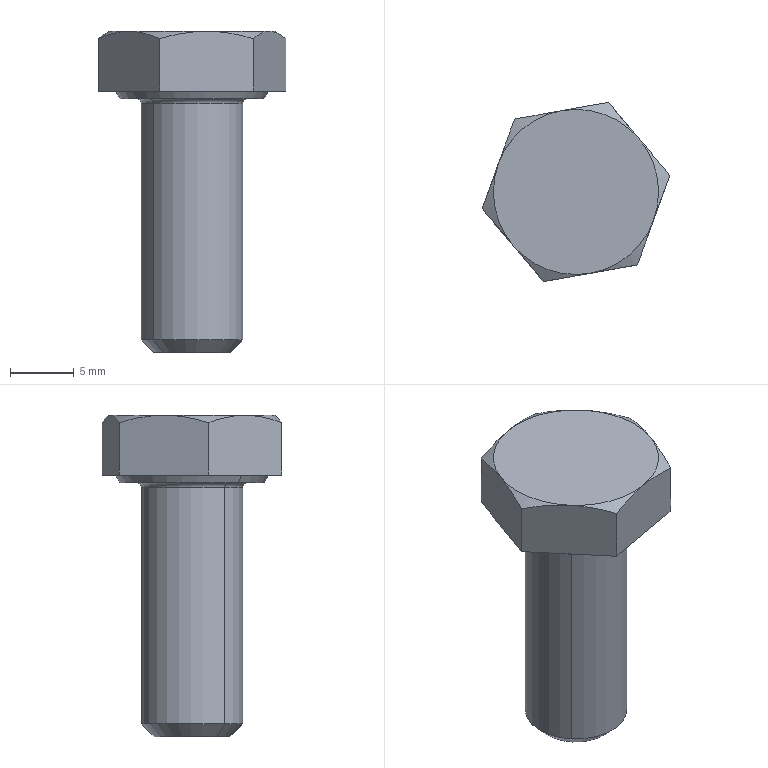Component | SolidWorks | GB_T5781-2000[HexHeadBoltFullThreadGradeCM8_20]-2 | 1 solid | 24 faces | box 14.78 x 14.12 x 25.3 mm | volume 1745 mm3 | cone 10 | plane 10 | cylinder 2 | torus 2 | commonest cylinder face diameters 8 x2
STEP:
#1=COLOUR_RGB('',0.7922,0.8196,0.9333);
#2=FILL_AREA_STYLE_COLOUR('',#1);
#3=FILL_AREA_STYLE('',(#2));
#4=SURFACE_STYLE_FILL_AREA(#3);
#5=SURFACE_SIDE_STYLE('',(#4));
#6=SURFACE_STYLE_USAGE(.BOTH.,#5);
#7=PRESENTATION_STYLE_ASSIGNMENT((#6));
#8=CARTESIAN_POINT('',(19.172,-21.185,97.148));
#9=VERTEX_POINT('',#8);
#10=CARTESIAN_POINT('',(18.931,-21.388,97.148));
#11=VERTEX_POINT('',#10);
#12=CARTESIAN_POINT('',(19.052,-21.287,97.148));
#13=DIRECTION('',(-0.,-0.,1.));
#14=DIRECTION('',(0.7644,0.6448,0.));
#15=AXIS2_PLACEMENT_3D('',#12,#13,#14);
#16=CIRCLE('',#15,0.1575);
#17=EDGE_CURVE('',#9,#11,#16,.T.);
#18=ORIENTED_EDGE('',*,*,#17,.F.);
#19=CARTESIAN_POINT('',(19.172,-21.185,96.416));
#20=VERTEX_POINT('',#19);
#21=CARTESIAN_POINT('',(19.172,-21.185,97.373));
#22=DIRECTION('',(0.,0.,-1.));
#23=VECTOR('',#22,39.37);
#24=LINE('',#21,#23);
#25=EDGE_CURVE('',#9,#20,#24,.T.);
#26=ORIENTED_EDGE('',*,*,#25,.T.);
#27=CARTESIAN_POINT('',(18.931,-21.388,96.416));
#28=VERTEX_POINT('',#27);
#29=CARTESIAN_POINT('',(19.052,-21.287,96.416));
#30=DIRECTION('',(-0.,-0.,1.));
#31=DIRECTION('',(-0.7644,-0.6448,-0.));
#32=AXIS2_PLACEMENT_3D('',#29,#30,#31);
#33=CIRCLE('',#32,0.1575);
#34=EDGE_CURVE('',#20,#28,#33,.T.);
#35=ORIENTED_EDGE('',*,*,#34,.T.);
#36=CARTESIAN_POINT('',(18.931,-21.388,97.373));
#37=DIRECTION('',(0.,0.,-1.));
#38=VECTOR('',#37,39.37);
#39=LINE('',#36,#38);
#40=EDGE_CURVE('',#11,#28,#39,.T.);
#41=ORIENTED_EDGE('',*,*,#40,.F.);
#42=EDGE_LOOP('',(#18,#26,#35,#41));
#43=FACE_OUTER_BOUND('',#42,.T.);
#44=CARTESIAN_POINT('',(19.052,-21.287,97.373));
#45=DIRECTION('',(0.,0.,-1.));
#46=DIRECTION('',(-0.7644,-0.6448,-0.));
#47=AXIS2_PLACEMENT_3D('',#44,#45,#46);
#48=CYLINDRICAL_SURFACE('',#47,0.1575);
#49=ADVANCED_FACE('',(#43),#48,.T.);
#50=CARTESIAN_POINT('',(18.962,-21.363,96.377));
#51=VERTEX_POINT('',#50);
#52=CARTESIAN_POINT('',(19.142,-21.21,96.377));
#53=VERTEX_POINT('',#52);
#54=CARTESIAN_POINT('',(19.052,-21.287,96.377));
#55=DIRECTION('',(0.,0.,-1.));
#56=DIRECTION('',(-0.7644,-0.6448,-0.));
#57=AXIS2_PLACEMENT_3D('',#54,#55,#56);
#58=CIRCLE('',#57,0.1181);
#59=EDGE_CURVE('',#51,#53,#58,.T.);
#60=ORIENTED_EDGE('',*,*,#59,.F.);
#61=CARTESIAN_POINT('',(18.962,-21.363,96.377));
#62=DIRECTION('',(-0.5405,-0.4559,0.7071));
#63=VECTOR('',#62,39.37);
#64=LINE('',#61,#63);
#65=EDGE_CURVE('',#51,#28,#64,.T.);
#66=ORIENTED_EDGE('',*,*,#65,.T.);
#67=ORIENTED_EDGE('',*,*,#34,.F.);
#68=CARTESIAN_POINT('',(19.142,-21.21,96.377));
#69=DIRECTION('',(0.5405,0.4559,0.7071));
#70=VECTOR('',#69,39.37);
#71=LINE('',#68,#70);
#72=EDGE_CURVE('',#53,#20,#71,.T.);
#73=ORIENTED_EDGE('',*,*,#72,.F.);
#74=EDGE_LOOP('',(#60,#66,#67,#73));
#75=FACE_OUTER_BOUND('',#74,.T.);
#76=CARTESIAN_POINT('',(19.052,-21.287,96.377));
#77=DIRECTION('',(-0.,-0.,1.));
#78=DIRECTION('',(0.7644,0.6448,0.));
#79=AXIS2_PLACEMENT_3D('',#76,#77,#78);
#80=CONICAL_SURFACE('',#79,0.1181,0.7854);
#81=ADVANCED_FACE('',(#75),#80,.T.);
#82=CARTESIAN_POINT('',(18.919,-21.398,97.164));
#83=VERTEX_POINT('',#82);
#84=CARTESIAN_POINT('',(19.184,-21.175,97.164));
#85=VERTEX_POINT('',#84);
#86=CARTESIAN_POINT('',(19.052,-21.287,97.164));
#87=DIRECTION('',(-0.,-0.,1.));
#88=DIRECTION('',(0.7644,0.6448,0.));
#89=AXIS2_PLACEMENT_3D('',#86,#87,#88);
#90=CIRCLE('',#89,0.1732);
#91=EDGE_CURVE('',#83,#85,#90,.T.);
#92=ORIENTED_EDGE('',*,*,#91,.F.);
#93=CARTESIAN_POINT('',(18.919,-21.398,97.148));
#94=DIRECTION('',(-0.6448,0.7644,0.));
#95=DIRECTION('',(-0.7644,-0.6448,0.));
#96=AXIS2_PLACEMENT_3D('',#93,#94,#95);
#97=CIRCLE('',#96,0.01575);
#98=EDGE_CURVE('',#83,#11,#97,.T.);
#99=ORIENTED_EDGE('',*,*,#98,.T.);
#100=CARTESIAN_POINT('',(19.052,-21.287,97.148));
#101=DIRECTION('',(-0.,-0.,1.));
#102=DIRECTION('',(0.7644,0.6448,0.));
#103=AXIS2_PLACEMENT_3D('',#100,#101,#102);
#104=CIRCLE('',#103,0.1575);
#105=EDGE_CURVE('',#11,#9,#104,.T.);
#106=ORIENTED_EDGE('',*,*,#105,.T.);
#107=CARTESIAN_POINT('',(19.184,-21.175,97.148));
#108=DIRECTION('',(0.6448,-0.7644,-0.));
#109=DIRECTION('',(0.7644,0.6448,0.));
#110=AXIS2_PLACEMENT_3D('',#107,#108,#109);
#111=CIRCLE('',#110,0.01575);
#112=EDGE_CURVE('',#85,#9,#111,.T.);
#113=ORIENTED_EDGE('',*,*,#112,.F.);
#114=EDGE_LOOP('',(#92,#99,#106,#113));
#115=FACE_OUTER_BOUND('',#114,.T.);
#116=CARTESIAN_POINT('',(19.052,-21.287,97.148));
#117=DIRECTION('',(-0.,-0.,1.));
#118=DIRECTION('',(0.7644,0.6448,0.));
#119=AXIS2_PLACEMENT_3D('',#116,#117,#118);
#120=TOROIDAL_SURFACE('',#119,0.1732,0.01575);
#121=ADVANCED_FACE('',(#115),#120,.F.);
#122=CARTESIAN_POINT('',(19.223,-21.143,97.164));
#123=VERTEX_POINT('',#122);
#124=CARTESIAN_POINT('',(18.881,-21.431,97.164));
#125=VERTEX_POINT('',#124);
#126=CARTESIAN_POINT('',(19.052,-21.287,97.164));
#127=DIRECTION('',(-0.,-0.,1.));
#128=DIRECTION('',(0.7644,0.6448,0.));
#129=AXIS2_PLACEMENT_3D('',#126,#127,#128);
#130=CIRCLE('',#129,0.2235);
#131=EDGE_CURVE('',#123,#125,#130,.T.);
#132=ORIENTED_EDGE('',*,*,#131,.T.);
#133=CARTESIAN_POINT('',(18.871,-21.44,97.188));
#134=VERTEX_POINT('',#133);
#135=CARTESIAN_POINT('',(18.871,-21.44,97.188));
#136=DIRECTION('',(-0.3822,-0.3224,0.866));
#137=VECTOR('',#136,39.37);
#138=LINE('',#135,#137);
#139=EDGE_CURVE('',#125,#134,#138,.T.);
#140=ORIENTED_EDGE('',*,*,#139,.T.);
#141=CARTESIAN_POINT('',(19.233,-21.134,97.188));
#142=VERTEX_POINT('',#141);
#143=CARTESIAN_POINT('',(19.052,-21.287,97.188));
#144=DIRECTION('',(-0.,-0.,1.));
#145=DIRECTION('',(0.7644,0.6448,0.));
#146=AXIS2_PLACEMENT_3D('',#143,#144,#145);
#147=CIRCLE('',#146,0.2372);
#148=EDGE_CURVE('',#142,#134,#147,.T.);
#149=ORIENTED_EDGE('',*,*,#148,.F.);
#150=CARTESIAN_POINT('',(19.233,-21.134,97.188));
#151=DIRECTION('',(0.3822,0.3224,0.866));
#152=VECTOR('',#151,39.37);
#153=LINE('',#150,#152);
#154=EDGE_CURVE('',#123,#142,#153,.T.);
#155=ORIENTED_EDGE('',*,*,#154,.F.);
#156=EDGE_LOOP('',(#132,#140,#149,#155));
#157=FACE_OUTER_BOUND('',#156,.T.);
#158=CARTESIAN_POINT('',(19.052,-21.287,97.188));
#159=DIRECTION('',(-0.,-0.,1.));
#160=DIRECTION('',(0.7644,0.6448,0.));
#161=AXIS2_PLACEMENT_3D('',#158,#159,#160);
#162=CONICAL_SURFACE('',#161,0.2372,0.5236);
#163=ADVANCED_FACE('',(#157),#162,.T.);
#164=ORIENTED_EDGE('',*,*,#131,.F.);
#165=CARTESIAN_POINT('',(19.052,-21.287,97.164));
#166=DIRECTION('',(-0.,-0.,1.));
#167=DIRECTION('',(0.7644,0.6448,0.));
#168=AXIS2_PLACEMENT_3D('',#165,#166,#167);
#169=CIRCLE('',#168,0.2235);
#170=EDGE_CURVE('',#125,#123,#169,.T.);
#171=ORIENTED_EDGE('',*,*,#170,.F.);
#172=EDGE_LOOP('',(#164,#171));
#173=FACE_OUTER_BOUND('',#172,.T.);
#174=CARTESIAN_POINT('',(19.052,-21.287,97.164));
#175=DIRECTION('',(-0.,-0.,1.));
#176=DIRECTION('',(0.7644,0.6448,0.));
#177=AXIS2_PLACEMENT_3D('',#174,#175,#176);
#178=CIRCLE('',#177,0.1732);
#179=EDGE_CURVE('',#85,#83,#178,.T.);
#180=ORIENTED_EDGE('',*,*,#179,.T.);
#181=ORIENTED_EDGE('',*,*,#91,.T.);
#182=EDGE_LOOP('',(#180,#181));
#183=FACE_BOUND('',#182,.T.);
#184=CARTESIAN_POINT('',(18.861,-21.061,97.164));
#185=DIRECTION('',(0.,0.,-1.));
#186=DIRECTION('',(-0.7644,-0.6448,-0.));
#187=AXIS2_PLACEMENT_3D('',#184,#185,#186);
#188=PLANE('',#187);
#189=ADVANCED_FACE('',(#173,#183),#188,.T.);
#190=CARTESIAN_POINT('',(18.761,-21.339,97.188));
#191=VERTEX_POINT('',#190);
#192=CARTESIAN_POINT('',(18.861,-21.061,97.188));
#193=VERTEX_POINT('',#192);
#194=CARTESIAN_POINT('',(18.761,-21.339,97.188));
#195=DIRECTION('',(0.3396,0.9406,0.));
#196=VECTOR('',#195,39.37);
#197=LINE('',#194,#196);
#198=EDGE_CURVE('',#191,#193,#197,.T.);
#199=ORIENTED_EDGE('',*,*,#198,.F.);
#200=CARTESIAN_POINT('',(18.761,-21.339,97.35));
#201=VERTEX_POINT('',#200);
#202=CARTESIAN_POINT('',(18.761,-21.339,97.164));
#203=DIRECTION('',(-0.,-0.,1.));
#204=VECTOR('',#203,39.37);
#205=LINE('',#202,#204);
#206=EDGE_CURVE('',#191,#201,#205,.T.);
#207=ORIENTED_EDGE('',*,*,#206,.T.);
#208=CARTESIAN_POINT('',(18.811,-21.2,97.373));
#209=VERTEX_POINT('',#208);
#210=CARTESIAN_POINT('',(18.811,-21.2,97.373));
#211=CARTESIAN_POINT('',(18.807,-21.212,97.373));
#212=CARTESIAN_POINT('',(18.803,-21.223,97.372));
#213=CARTESIAN_POINT('',(18.794,-21.247,97.37));
#214=CARTESIAN_POINT('',(18.79,-21.258,97.369));
#215=CARTESIAN_POINT('',(18.777,-21.293,97.363));
#216=CARTESIAN_POINT('',(18.769,-21.316,97.357));
#217=CARTESIAN_POINT('',(18.761,-21.339,97.35));
#218=B_SPLINE_CURVE_WITH_KNOTS('',3,(#210,#211,#212,#213,#214,#215,#216,#217),.UNSPECIFIED.,.F.,.F.,(4,2,2,4),(0.003797,0.004743,0.005689,0.00758),.UNSPECIFIED.);
#219=EDGE_CURVE('',#209,#201,#218,.T.);
#220=ORIENTED_EDGE('',*,*,#219,.F.);
#221=CARTESIAN_POINT('',(18.861,-21.061,97.35));
#222=VERTEX_POINT('',#221);
#223=CARTESIAN_POINT('',(18.861,-21.061,97.35));
#224=CARTESIAN_POINT('',(18.853,-21.084,97.357));
#225=CARTESIAN_POINT('',(18.845,-21.106,97.363));
#226=CARTESIAN_POINT('',(18.828,-21.153,97.371));
#227=CARTESIAN_POINT('',(18.82,-21.176,97.373));
#228=CARTESIAN_POINT('',(18.811,-21.2,97.373));
#229=B_SPLINE_CURVE_WITH_KNOTS('',3,(#223,#224,#225,#226,#227,#228),.UNSPECIFIED.,.F.,.F.,(4,2,4),(0.00000024,0.001899,0.003797),.UNSPECIFIED.);
#230=EDGE_CURVE('',#222,#209,#229,.T.);
#231=ORIENTED_EDGE('',*,*,#230,.F.);
#232=CARTESIAN_POINT('',(18.861,-21.061,97.164));
#233=DIRECTION('',(-0.,-0.,1.));
#234=VECTOR('',#233,39.37);
#235=LINE('',#232,#234);
#236=EDGE_CURVE('',#193,#222,#235,.T.);
#237=ORIENTED_EDGE('',*,*,#236,.F.);
#238=EDGE_LOOP('',(#199,#207,#220,#231,#237));
#239=FACE_OUTER_BOUND('',#238,.T.);
#240=CARTESIAN_POINT('',(18.761,-21.339,97.164));
#241=DIRECTION('',(0.9406,-0.3396,-0.));
#242=DIRECTION('',(-0.3396,-0.9406,-0.));
#243=AXIS2_PLACEMENT_3D('',#240,#241,#242);
#244=PLANE('',#243);
#245=ADVANCED_FACE('',(#239),#244,.F.);
#246=CARTESIAN_POINT('',(19.152,-21.009,97.188));
#247=VERTEX_POINT('',#246);
#248=CARTESIAN_POINT('',(18.861,-21.061,97.188));
#249=DIRECTION('',(0.9844,0.1762,0.));
#250=VECTOR('',#249,39.37);
#251=LINE('',#248,#250);
#252=EDGE_CURVE('',#193,#247,#251,.T.);
#253=ORIENTED_EDGE('',*,*,#252,.F.);
#254=ORIENTED_EDGE('',*,*,#236,.T.);
#255=CARTESIAN_POINT('',(19.007,-21.035,97.373));
#256=VERTEX_POINT('',#255);
#257=CARTESIAN_POINT('',(19.007,-21.035,97.373));
#258=CARTESIAN_POINT('',(18.994,-21.037,97.373));
#259=CARTESIAN_POINT('',(18.982,-21.039,97.372));
#260=CARTESIAN_POINT('',(18.957,-21.044,97.37));
#261=CARTESIAN_POINT('',(18.945,-21.046,97.369));
#262=CARTESIAN_POINT('',(18.909,-21.052,97.363));
#263=CARTESIAN_POINT('',(18.885,-21.057,97.357));
#264=CARTESIAN_POINT('',(18.861,-21.061,97.35));
#265=B_SPLINE_CURVE_WITH_KNOTS('',3,(#257,#258,#259,#260,#261,#262,#263,#264),.UNSPECIFIED.,.F.,.F.,(4,2,2,4),(0.003797,0.004743,0.005689,0.00758),.UNSPECIFIED.);
#266=EDGE_CURVE('',#256,#222,#265,.T.);
#267=ORIENTED_EDGE('',*,*,#266,.F.);
#268=CARTESIAN_POINT('',(19.152,-21.009,97.35));
#269=VERTEX_POINT('',#268);
#270=CARTESIAN_POINT('',(19.152,-21.009,97.35));
#271=CARTESIAN_POINT('',(19.128,-21.013,97.357));
#272=CARTESIAN_POINT('',(19.104,-21.017,97.363));
#273=CARTESIAN_POINT('',(19.056,-21.026,97.371));
#274=CARTESIAN_POINT('',(19.032,-21.03,97.373));
#275=CARTESIAN_POINT('',(19.007,-21.035,97.373));
#276=B_SPLINE_CURVE_WITH_KNOTS('',3,(#270,#271,#272,#273,#274,#275),.UNSPECIFIED.,.F.,.F.,(4,2,4),(0.00000024,0.001899,0.003797),.UNSPECIFIED.);
#277=EDGE_CURVE('',#269,#256,#276,.T.);
#278=ORIENTED_EDGE('',*,*,#277,.F.);
#279=CARTESIAN_POINT('',(19.152,-21.009,97.164));
#280=DIRECTION('',(-0.,-0.,1.));
#281=VECTOR('',#280,39.37);
#282=LINE('',#279,#281);
#283=EDGE_CURVE('',#247,#269,#282,.T.);
#284=ORIENTED_EDGE('',*,*,#283,.F.);
#285=EDGE_LOOP('',(#253,#254,#267,#278,#284));
#286=FACE_OUTER_BOUND('',#285,.T.);
#287=CARTESIAN_POINT('',(18.861,-21.061,97.164));
#288=DIRECTION('',(0.1762,-0.9844,-0.));
#289=DIRECTION('',(-0.9844,-0.1762,-0.));
#290=AXIS2_PLACEMENT_3D('',#287,#288,#289);
#291=PLANE('',#290);
#292=ADVANCED_FACE('',(#286),#291,.F.);
#293=CARTESIAN_POINT('',(19.343,-21.235,97.188));
#294=VERTEX_POINT('',#293);
#295=CARTESIAN_POINT('',(19.152,-21.009,97.188));
#296=DIRECTION('',(0.6448,-0.7644,-0.));
#297=VECTOR('',#296,39.37);
#298=LINE('',#295,#297);
#299=EDGE_CURVE('',#247,#294,#298,.T.);
#300=ORIENTED_EDGE('',*,*,#299,.F.);
#301=ORIENTED_EDGE('',*,*,#283,.T.);
#302=CARTESIAN_POINT('',(19.247,-21.122,97.373));
#303=VERTEX_POINT('',#302);
#304=CARTESIAN_POINT('',(19.247,-21.122,97.373));
#305=CARTESIAN_POINT('',(19.231,-21.103,97.373));
#306=CARTESIAN_POINT('',(19.215,-21.083,97.371));
#307=CARTESIAN_POINT('',(19.183,-21.045,97.363));
#308=CARTESIAN_POINT('',(19.168,-21.027,97.357));
#309=CARTESIAN_POINT('',(19.152,-21.009,97.35));
#310=B_SPLINE_CURVE_WITH_KNOTS('',3,(#304,#305,#306,#307,#308,#309),.UNSPECIFIED.,.F.,.F.,(4,2,4),(0.01067,0.01257,0.01447),.UNSPECIFIED.);
#311=EDGE_CURVE('',#303,#269,#310,.T.);
#312=ORIENTED_EDGE('',*,*,#311,.F.);
#313=CARTESIAN_POINT('',(19.343,-21.235,97.35));
#314=VERTEX_POINT('',#313);
#315=CARTESIAN_POINT('',(19.343,-21.235,97.35));
#316=CARTESIAN_POINT('',(19.327,-21.216,97.357));
#317=CARTESIAN_POINT('',(19.311,-21.197,97.363));
#318=CARTESIAN_POINT('',(19.28,-21.16,97.371));
#319=CARTESIAN_POINT('',(19.264,-21.141,97.373));
#320=CARTESIAN_POINT('',(19.247,-21.122,97.373));
#321=B_SPLINE_CURVE_WITH_KNOTS('',3,(#315,#316,#317,#318,#319,#320),.UNSPECIFIED.,.F.,.F.,(4,2,4),(0.006874,0.008773,0.01067),.UNSPECIFIED.);
#322=EDGE_CURVE('',#314,#303,#321,.T.);
#323=ORIENTED_EDGE('',*,*,#322,.F.);
#324=CARTESIAN_POINT('',(19.343,-21.235,97.164));
#325=DIRECTION('',(-0.,-0.,1.));
#326=VECTOR('',#325,39.37);
#327=LINE('',#324,#326);
#328=EDGE_CURVE('',#294,#314,#327,.T.);
#329=ORIENTED_EDGE('',*,*,#328,.F.);
#330=EDGE_LOOP('',(#300,#301,#312,#323,#329));
#331=FACE_OUTER_BOUND('',#330,.T.);
#332=CARTESIAN_POINT('',(19.152,-21.009,97.164));
#333=DIRECTION('',(-0.7644,-0.6448,-0.));
#334=DIRECTION('',(-0.6448,0.7644,0.));
#335=AXIS2_PLACEMENT_3D('',#332,#333,#334);
#336=PLANE('',#335);
#337=ADVANCED_FACE('',(#331),#336,.F.);
#338=CARTESIAN_POINT('',(19.242,-21.513,97.188));
#339=VERTEX_POINT('',#338);
#340=CARTESIAN_POINT('',(19.242,-21.513,97.188));
#341=DIRECTION('',(-0.3396,-0.9406,-0.));
#342=VECTOR('',#341,39.37);
#343=LINE('',#340,#342);
#344=EDGE_CURVE('',#294,#339,#343,.T.);
#345=ORIENTED_EDGE('',*,*,#344,.F.);
#346=ORIENTED_EDGE('',*,*,#328,.T.);
#347=CARTESIAN_POINT('',(19.293,-21.374,97.373));
#348=VERTEX_POINT('',#347);
#349=CARTESIAN_POINT('',(19.293,-21.374,97.373));
#350=CARTESIAN_POINT('',(19.297,-21.362,97.373));
#351=CARTESIAN_POINT('',(19.301,-21.35,97.372));
#352=CARTESIAN_POINT('',(19.31,-21.326,97.37));
#353=CARTESIAN_POINT('',(19.314,-21.315,97.369));
#354=CARTESIAN_POINT('',(19.326,-21.28,97.363));
#355=CARTESIAN_POINT('',(19.335,-21.257,97.357));
#356=CARTESIAN_POINT('',(19.343,-21.235,97.35));
#357=B_SPLINE_CURVE_WITH_KNOTS('',3,(#349,#350,#351,#352,#353,#354,#355,#356),.UNSPECIFIED.,.F.,.F.,(4,2,2,4),(0.003797,0.004743,0.005689,0.00758),.UNSPECIFIED.);
#358=EDGE_CURVE('',#348,#314,#357,.T.);
#359=ORIENTED_EDGE('',*,*,#358,.F.);
#360=CARTESIAN_POINT('',(19.242,-21.513,97.35));
#361=VERTEX_POINT('',#360);
#362=CARTESIAN_POINT('',(19.242,-21.513,97.35));
#363=CARTESIAN_POINT('',(19.251,-21.49,97.357));
#364=CARTESIAN_POINT('',(19.259,-21.467,97.363));
#365=CARTESIAN_POINT('',(19.276,-21.421,97.371));
#366=CARTESIAN_POINT('',(19.284,-21.397,97.373));
#367=CARTESIAN_POINT('',(19.293,-21.374,97.373));
#368=B_SPLINE_CURVE_WITH_KNOTS('',3,(#362,#363,#364,#365,#366,#367),.UNSPECIFIED.,.F.,.F.,(4,2,4),(0.00000024,0.001899,0.003797),.UNSPECIFIED.);
#369=EDGE_CURVE('',#361,#348,#368,.T.);
#370=ORIENTED_EDGE('',*,*,#369,.F.);
#371=CARTESIAN_POINT('',(19.242,-21.513,97.164));
#372=DIRECTION('',(-0.,-0.,1.));
#373=VECTOR('',#372,39.37);
#374=LINE('',#371,#373);
#375=EDGE_CURVE('',#339,#361,#374,.T.);
#376=ORIENTED_EDGE('',*,*,#375,.F.);
#377=EDGE_LOOP('',(#345,#346,#359,#370,#376));
#378=FACE_OUTER_BOUND('',#377,.T.);
#379=CARTESIAN_POINT('',(19.242,-21.513,97.164));
#380=DIRECTION('',(-0.9406,0.3396,0.));
#381=DIRECTION('',(0.3396,0.9406,0.));
#382=AXIS2_PLACEMENT_3D('',#379,#380,#381);
#383=PLANE('',#382);
#384=ADVANCED_FACE('',(#378),#383,.F.);
#385=CARTESIAN_POINT('',(18.951,-21.565,97.188));
#386=VERTEX_POINT('',#385);
#387=CARTESIAN_POINT('',(18.951,-21.565,97.188));
#388=DIRECTION('',(-0.9844,-0.1762,-0.));
#389=VECTOR('',#388,39.37);
#390=LINE('',#387,#389);
#391=EDGE_CURVE('',#339,#386,#390,.T.);
#392=ORIENTED_EDGE('',*,*,#391,.F.);
#393=ORIENTED_EDGE('',*,*,#375,.T.);
#394=CARTESIAN_POINT('',(19.097,-21.539,97.373));
#395=VERTEX_POINT('',#394);
#396=CARTESIAN_POINT('',(19.097,-21.539,97.373));
#397=CARTESIAN_POINT('',(19.109,-21.536,97.373));
#398=CARTESIAN_POINT('',(19.122,-21.534,97.372));
#399=CARTESIAN_POINT('',(19.146,-21.53,97.37));
#400=CARTESIAN_POINT('',(19.158,-21.528,97.369));
#401=CARTESIAN_POINT('',(19.195,-21.521,97.363));
#402=CARTESIAN_POINT('',(19.219,-21.517,97.357));
#403=CARTESIAN_POINT('',(19.242,-21.513,97.35));
#404=B_SPLINE_CURVE_WITH_KNOTS('',3,(#396,#397,#398,#399,#400,#401,#402,#403),.UNSPECIFIED.,.F.,.F.,(4,2,2,4),(0.003797,0.004743,0.005689,0.00758),.UNSPECIFIED.);
#405=EDGE_CURVE('',#395,#361,#404,.T.);
#406=ORIENTED_EDGE('',*,*,#405,.F.);
#407=CARTESIAN_POINT('',(18.951,-21.565,97.35));
#408=VERTEX_POINT('',#407);
#409=CARTESIAN_POINT('',(18.951,-21.565,97.35));
#410=CARTESIAN_POINT('',(18.975,-21.56,97.357));
#411=CARTESIAN_POINT('',(18.999,-21.556,97.363));
#412=CARTESIAN_POINT('',(19.048,-21.547,97.371));
#413=CARTESIAN_POINT('',(19.072,-21.543,97.373));
#414=CARTESIAN_POINT('',(19.097,-21.539,97.373));
#415=B_SPLINE_CURVE_WITH_KNOTS('',3,(#409,#410,#411,#412,#413,#414),.UNSPECIFIED.,.F.,.F.,(4,2,4),(0.00000024,0.001899,0.003797),.UNSPECIFIED.);
#416=EDGE_CURVE('',#408,#395,#415,.T.);
#417=ORIENTED_EDGE('',*,*,#416,.F.);
#418=CARTESIAN_POINT('',(18.951,-21.565,97.164));
#419=DIRECTION('',(-0.,-0.,1.));
#420=VECTOR('',#419,39.37);
#421=LINE('',#418,#420);
#422=EDGE_CURVE('',#386,#408,#421,.T.);
#423=ORIENTED_EDGE('',*,*,#422,.F.);
#424=EDGE_LOOP('',(#392,#393,#406,#417,#423));
#425=FACE_OUTER_BOUND('',#424,.T.);
#426=CARTESIAN_POINT('',(18.951,-21.565,97.164));
#427=DIRECTION('',(-0.1762,0.9844,0.));
#428=DIRECTION('',(0.9844,0.1762,0.));
#429=AXIS2_PLACEMENT_3D('',#426,#427,#428);
#430=PLANE('',#429);
#431=ADVANCED_FACE('',(#425),#430,.F.);
#432=CARTESIAN_POINT('',(18.761,-21.339,97.188));
#433=DIRECTION('',(-0.6448,0.7644,0.));
#434=VECTOR('',#433,39.37);
#435=LINE('',#432,#434);
#436=EDGE_CURVE('',#386,#191,#435,.T.);
#437=ORIENTED_EDGE('',*,*,#436,.F.);
#438=ORIENTED_EDGE('',*,*,#422,.T.);
#439=CARTESIAN_POINT('',(18.856,-21.452,97.373));
#440=VERTEX_POINT('',#439);
#441=CARTESIAN_POINT('',(18.856,-21.452,97.373));
#442=CARTESIAN_POINT('',(18.872,-21.471,97.373));
#443=CARTESIAN_POINT('',(18.888,-21.49,97.371));
#444=CARTESIAN_POINT('',(18.92,-21.527,97.363));
#445=CARTESIAN_POINT('',(18.936,-21.546,97.357));
#446=CARTESIAN_POINT('',(18.951,-21.565,97.35));
#447=B_SPLINE_CURVE_WITH_KNOTS('',3,(#441,#442,#443,#444,#445,#446),.UNSPECIFIED.,.F.,.F.,(4,2,4),(0.02294,0.02484,0.02674),.UNSPECIFIED.);
#448=EDGE_CURVE('',#440,#408,#447,.T.);
#449=ORIENTED_EDGE('',*,*,#448,.F.);
#450=CARTESIAN_POINT('',(18.761,-21.339,97.35));
#451=CARTESIAN_POINT('',(18.776,-21.357,97.357));
#452=CARTESIAN_POINT('',(18.792,-21.375,97.363));
#453=CARTESIAN_POINT('',(18.824,-21.413,97.371));
#454=CARTESIAN_POINT('',(18.84,-21.433,97.373));
#455=CARTESIAN_POINT('',(18.856,-21.452,97.373));
#456=B_SPLINE_CURVE_WITH_KNOTS('',3,(#450,#451,#452,#453,#454,#455),.UNSPECIFIED.,.F.,.F.,(4,2,4),(0.01914,0.02104,0.02294),.UNSPECIFIED.);
#457=EDGE_CURVE('',#201,#440,#456,.T.);
#458=ORIENTED_EDGE('',*,*,#457,.F.);
#459=ORIENTED_EDGE('',*,*,#206,.F.);
#460=EDGE_LOOP('',(#437,#438,#449,#458,#459));
#461=FACE_OUTER_BOUND('',#460,.T.);
#462=CARTESIAN_POINT('',(18.761,-21.339,97.164));
#463=DIRECTION('',(0.7644,0.6448,0.));
#464=DIRECTION('',(0.6448,-0.7644,-0.));
#465=AXIS2_PLACEMENT_3D('',#462,#463,#464);
#466=PLANE('',#465);
#467=ADVANCED_FACE('',(#461),#466,.F.);
#468=ORIENTED_EDGE('',*,*,#416,.T.);
#469=CARTESIAN_POINT('',(19.052,-21.287,97.373));
#470=DIRECTION('',(0.,0.,-1.));
#471=DIRECTION('',(-0.7644,-0.6448,-0.));
#472=AXIS2_PLACEMENT_3D('',#469,#470,#471);
#473=CIRCLE('',#472,0.2559);
#474=EDGE_CURVE('',#395,#440,#473,.T.);
#475=ORIENTED_EDGE('',*,*,#474,.T.);
#476=ORIENTED_EDGE('',*,*,#448,.T.);
#477=EDGE_LOOP('',(#468,#475,#476));
#478=FACE_OUTER_BOUND('',#477,.T.);
#479=CARTESIAN_POINT('',(19.052,-21.287,97.373));
#480=DIRECTION('',(0.,0.,-1.));
#481=DIRECTION('',(-0.7644,-0.6448,-0.));
#482=AXIS2_PLACEMENT_3D('',#479,#480,#481);
#483=CONICAL_SURFACE('',#482,0.2559,1.047);
#484=ADVANCED_FACE('',(#478),#483,.T.);
#485=ORIENTED_EDGE('',*,*,#369,.T.);
#486=CARTESIAN_POINT('',(19.052,-21.287,97.373));
#487=DIRECTION('',(0.,0.,-1.));
#488=DIRECTION('',(-0.7644,-0.6448,-0.));
#489=AXIS2_PLACEMENT_3D('',#486,#487,#488);
#490=CIRCLE('',#489,0.2559);
#491=EDGE_CURVE('',#348,#395,#490,.T.);
#492=ORIENTED_EDGE('',*,*,#491,.T.);
#493=ORIENTED_EDGE('',*,*,#405,.T.);
#494=EDGE_LOOP('',(#485,#492,#493));
#495=FACE_OUTER_BOUND('',#494,.T.);
#496=CARTESIAN_POINT('',(19.052,-21.287,97.373));
#497=DIRECTION('',(0.,0.,-1.));
#498=DIRECTION('',(-0.7644,-0.6448,-0.));
#499=AXIS2_PLACEMENT_3D('',#496,#497,#498);
#500=CONICAL_SURFACE('',#499,0.2559,1.047);
#501=ADVANCED_FACE('',(#495),#500,.T.);
#502=ORIENTED_EDGE('',*,*,#322,.T.);
#503=CARTESIAN_POINT('',(19.052,-21.287,97.373));
#504=DIRECTION('',(0.,0.,-1.));
#505=DIRECTION('',(-0.7644,-0.6448,-0.));
#506=AXIS2_PLACEMENT_3D('',#503,#504,#505);
#507=CIRCLE('',#506,0.2559);
#508=EDGE_CURVE('',#303,#348,#507,.T.);
#509=ORIENTED_EDGE('',*,*,#508,.T.);
#510=ORIENTED_EDGE('',*,*,#358,.T.);
#511=EDGE_LOOP('',(#502,#509,#510));
#512=FACE_OUTER_BOUND('',#511,.T.);
#513=CARTESIAN_POINT('',(19.052,-21.287,97.373));
#514=DIRECTION('',(0.,0.,-1.));
#515=DIRECTION('',(-0.7644,-0.6448,-0.));
#516=AXIS2_PLACEMENT_3D('',#513,#514,#515);
#517=CONICAL_SURFACE('',#516,0.2559,1.047);
#518=ADVANCED_FACE('',(#512),#517,.T.);
#519=ORIENTED_EDGE('',*,*,#311,.T.);
#520=ORIENTED_EDGE('',*,*,#277,.T.);
#521=CARTESIAN_POINT('',(19.052,-21.287,97.373));
#522=DIRECTION('',(-0.,-0.,1.));
#523=DIRECTION('',(0.7644,0.6448,0.));
#524=AXIS2_PLACEMENT_3D('',#521,#522,#523);
#525=CIRCLE('',#524,0.2559);
#526=EDGE_CURVE('',#303,#256,#525,.T.);
#527=ORIENTED_EDGE('',*,*,#526,.F.);
#528=EDGE_LOOP('',(#519,#520,#527));
#529=FACE_OUTER_BOUND('',#528,.T.);
#530=CARTESIAN_POINT('',(19.052,-21.287,97.373));
#531=DIRECTION('',(0.,0.,-1.));
#532=DIRECTION('',(-0.7644,-0.6448,-0.));
#533=AXIS2_PLACEMENT_3D('',#530,#531,#532);
#534=CONICAL_SURFACE('',#533,0.2559,1.047);
#535=ADVANCED_FACE('',(#529),#534,.T.);
#536=ORIENTED_EDGE('',*,*,#266,.T.);
#537=ORIENTED_EDGE('',*,*,#230,.T.);
#538=CARTESIAN_POINT('',(19.052,-21.287,97.373));
#539=DIRECTION('',(0.,0.,-1.));
#540=DIRECTION('',(-0.7644,-0.6448,-0.));
#541=AXIS2_PLACEMENT_3D('',#538,#539,#540);
#542=CIRCLE('',#541,0.2559);
#543=EDGE_CURVE('',#209,#256,#542,.T.);
#544=ORIENTED_EDGE('',*,*,#543,.T.);
#545=EDGE_LOOP('',(#536,#537,#544));
#546=FACE_OUTER_BOUND('',#545,.T.);
#547=CARTESIAN_POINT('',(19.052,-21.287,97.373));
#548=DIRECTION('',(0.,0.,-1.));
#549=DIRECTION('',(-0.7644,-0.6448,-0.));
#550=AXIS2_PLACEMENT_3D('',#547,#548,#549);
#551=CONICAL_SURFACE('',#550,0.2559,1.047);
#552=ADVANCED_FACE('',(#546),#551,.T.);
#553=ORIENTED_EDGE('',*,*,#219,.T.);
#554=ORIENTED_EDGE('',*,*,#457,.T.);
#555=CARTESIAN_POINT('',(19.052,-21.287,97.373));
#556=DIRECTION('',(0.,0.,-1.));
#557=DIRECTION('',(-0.7644,-0.6448,-0.));
#558=AXIS2_PLACEMENT_3D('',#555,#556,#557);
#559=CIRCLE('',#558,0.2559);
#560=EDGE_CURVE('',#440,#209,#559,.T.);
#561=ORIENTED_EDGE('',*,*,#560,.T.);
#562=EDGE_LOOP('',(#553,#554,#561));
#563=FACE_OUTER_BOUND('',#562,.T.);
#564=CARTESIAN_POINT('',(19.052,-21.287,97.373));
#565=DIRECTION('',(0.,0.,-1.));
#566=DIRECTION('',(-0.7644,-0.6448,-0.));
#567=AXIS2_PLACEMENT_3D('',#564,#565,#566);
#568=CONICAL_SURFACE('',#567,0.2559,1.047);
#569=ADVANCED_FACE('',(#563),#568,.T.);
#570=ORIENTED_EDGE('',*,*,#560,.F.);
#571=ORIENTED_EDGE('',*,*,#474,.F.);
#572=ORIENTED_EDGE('',*,*,#491,.F.);
#573=ORIENTED_EDGE('',*,*,#508,.F.);
#574=ORIENTED_EDGE('',*,*,#526,.T.);
#575=ORIENTED_EDGE('',*,*,#543,.F.);
#576=EDGE_LOOP('',(#570,#571,#572,#573,#574,#575));
#577=FACE_OUTER_BOUND('',#576,.T.);
#578=CARTESIAN_POINT('',(18.861,-21.061,97.373));
#579=DIRECTION('',(0.,0.,-1.));
#580=DIRECTION('',(-0.7644,-0.6448,-0.));
#581=AXIS2_PLACEMENT_3D('',#578,#579,#580);
#582=PLANE('',#581);
#583=ADVANCED_FACE('',(#577),#582,.F.);
#584=ORIENTED_EDGE('',*,*,#148,.T.);
#585=CARTESIAN_POINT('',(19.052,-21.287,97.188));
#586=DIRECTION('',(-0.,-0.,1.));
#587=DIRECTION('',(0.7644,0.6448,0.));
#588=AXIS2_PLACEMENT_3D('',#585,#586,#587);
#589=CIRCLE('',#588,0.2372);
#590=EDGE_CURVE('',#134,#142,#589,.T.);
#591=ORIENTED_EDGE('',*,*,#590,.T.);
#592=EDGE_LOOP('',(#584,#591));
#593=FACE_BOUND('',#592,.T.);
#594=ORIENTED_EDGE('',*,*,#198,.T.);
#595=ORIENTED_EDGE('',*,*,#252,.T.);
#596=ORIENTED_EDGE('',*,*,#299,.T.);
#597=ORIENTED_EDGE('',*,*,#344,.T.);
#598=ORIENTED_EDGE('',*,*,#391,.T.);
#599=ORIENTED_EDGE('',*,*,#436,.T.);
#600=EDGE_LOOP('',(#594,#595,#596,#597,#598,#599));
#601=FACE_OUTER_BOUND('',#600,.T.);
#602=CARTESIAN_POINT('',(18.899,-21.105,97.188));
#603=DIRECTION('',(0.,0.,-1.));
#604=DIRECTION('',(-0.7644,-0.6448,-0.));
#605=AXIS2_PLACEMENT_3D('',#602,#603,#604);
#606=PLANE('',#605);
#607=ADVANCED_FACE('',(#593,#601),#606,.T.);
#608=ORIENTED_EDGE('',*,*,#139,.F.);
#609=ORIENTED_EDGE('',*,*,#170,.T.);
#610=ORIENTED_EDGE('',*,*,#154,.T.);
#611=ORIENTED_EDGE('',*,*,#590,.F.);
#612=EDGE_LOOP('',(#608,#609,#610,#611));
#613=FACE_OUTER_BOUND('',#612,.T.);
#614=CARTESIAN_POINT('',(19.052,-21.287,97.188));
#615=DIRECTION('',(-0.,-0.,1.));
#616=DIRECTION('',(0.7644,0.6448,0.));
#617=AXIS2_PLACEMENT_3D('',#614,#615,#616);
#618=CONICAL_SURFACE('',#617,0.2372,0.5236);
#619=ADVANCED_FACE('',(#613),#618,.T.);
#620=ORIENTED_EDGE('',*,*,#98,.F.);
#621=ORIENTED_EDGE('',*,*,#179,.F.);
#622=ORIENTED_EDGE('',*,*,#112,.T.);
#623=ORIENTED_EDGE('',*,*,#17,.T.);
#624=EDGE_LOOP('',(#620,#621,#622,#623));
#625=FACE_OUTER_BOUND('',#624,.T.);
#626=CARTESIAN_POINT('',(19.052,-21.287,97.148));
#627=DIRECTION('',(-0.,-0.,1.));
#628=DIRECTION('',(0.7644,0.6448,0.));
#629=AXIS2_PLACEMENT_3D('',#626,#627,#628);
#630=TOROIDAL_SURFACE('',#629,0.1732,0.01575);
#631=ADVANCED_FACE('',(#625),#630,.F.);
#632=CARTESIAN_POINT('',(19.052,-21.287,96.377));
#633=DIRECTION('',(0.,0.,-1.));
#634=DIRECTION('',(-0.7644,-0.6448,-0.));
#635=AXIS2_PLACEMENT_3D('',#632,#633,#634);
#636=CIRCLE('',#635,0.1181);
#637=EDGE_CURVE('',#53,#51,#636,.T.);
#638=ORIENTED_EDGE('',*,*,#637,.T.);
#639=ORIENTED_EDGE('',*,*,#59,.T.);
#640=EDGE_LOOP('',(#638,#639));
#641=FACE_OUTER_BOUND('',#640,.T.);
#642=CARTESIAN_POINT('',(19.052,-21.287,96.377));
#643=DIRECTION('',(0.,0.,-1.));
#644=DIRECTION('',(-0.7644,-0.6448,-0.));
#645=AXIS2_PLACEMENT_3D('',#642,#643,#644);
#646=PLANE('',#645);
#647=ADVANCED_FACE('',(#641),#646,.T.);
#648=ORIENTED_EDGE('',*,*,#65,.F.);
#649=ORIENTED_EDGE('',*,*,#637,.F.);
#650=ORIENTED_EDGE('',*,*,#72,.T.);
#651=CARTESIAN_POINT('',(19.052,-21.287,96.416));
#652=DIRECTION('',(-0.,-0.,1.));
#653=DIRECTION('',(-0.7644,-0.6448,-0.));
#654=AXIS2_PLACEMENT_3D('',#651,#652,#653);
#655=CIRCLE('',#654,0.1575);
#656=EDGE_CURVE('',#28,#20,#655,.T.);
#657=ORIENTED_EDGE('',*,*,#656,.F.);
#658=EDGE_LOOP('',(#648,#649,#650,#657));
#659=FACE_OUTER_BOUND('',#658,.T.);
#660=CARTESIAN_POINT('',(19.052,-21.287,96.377));
#661=DIRECTION('',(-0.,-0.,1.));
#662=DIRECTION('',(0.7644,0.6448,0.));
#663=AXIS2_PLACEMENT_3D('',#660,#661,#662);
#664=CONICAL_SURFACE('',#663,0.1181,0.7854);
#665=ADVANCED_FACE('',(#659),#664,.T.);
#666=ORIENTED_EDGE('',*,*,#25,.F.);
#667=ORIENTED_EDGE('',*,*,#105,.F.);
#668=ORIENTED_EDGE('',*,*,#40,.T.);
#669=ORIENTED_EDGE('',*,*,#656,.T.);
#670=EDGE_LOOP('',(#666,#667,#668,#669));
#671=FACE_OUTER_BOUND('',#670,.T.);
#672=CARTESIAN_POINT('',(19.052,-21.287,97.373));
#673=DIRECTION('',(0.,0.,-1.));
#674=DIRECTION('',(-0.7644,-0.6448,-0.));
#675=AXIS2_PLACEMENT_3D('',#672,#673,#674);
#676=CYLINDRICAL_SURFACE('',#675,0.1575);
#677=ADVANCED_FACE('',(#671),#676,.T.);
#678=CLOSED_SHELL('',(#49,#81,#121,#163,#189,#245,#292,#337,#384,#431,#467,#484,#501,#518,#535,#552,#569,#583,#607,#619,#631,#647,#665,#677));
#679=MANIFOLD_SOLID_BREP('',#678);
#680=STYLED_ITEM('',(#7),#679);
#681=(LENGTH_UNIT()NAMED_UNIT(*)SI_UNIT($,.METRE.));
#682=LENGTH_MEASURE_WITH_UNIT(LENGTH_MEASURE(0.0254),#681);
#683=DIMENSIONAL_EXPONENTS(1.,0.,0.,0.,0.,0.,0.);
#684=(CONVERSION_BASED_UNIT('',#682)LENGTH_UNIT()NAMED_UNIT(#683));
#685=UNCERTAINTY_MEASURE_WITH_UNIT(LENGTH_MEASURE(0.00001),#684,'','');
#686=(NAMED_UNIT(*)PLANE_ANGLE_UNIT()SI_UNIT($,.RADIAN.));
#687=(NAMED_UNIT(*)SI_UNIT($,.STERADIAN.)SOLID_ANGLE_UNIT());
#688=(GEOMETRIC_REPRESENTATION_CONTEXT(3)GLOBAL_UNCERTAINTY_ASSIGNED_CONTEXT((#685))GLOBAL_UNIT_ASSIGNED_CONTEXT((#684,#686,#687))REPRESENTATION_CONTEXT('',''));
#689=MECHANICAL_DESIGN_GEOMETRIC_PRESENTATION_REPRESENTATION('',(#680),#688);
#690=PRESENTATION_LAYER_ASSIGNMENT('','',(#680));
#691=CARTESIAN_POINT('',(0.,0.,0.));
#692=DIRECTION('',(0.,0.,1.));
#693=DIRECTION('',(1.,0.,0.));
#694=AXIS2_PLACEMENT_3D('',#691,#692,#693);
#695=(LENGTH_UNIT()NAMED_UNIT(*)SI_UNIT($,.METRE.));
#696=LENGTH_MEASURE_WITH_UNIT(LENGTH_MEASURE(0.0254),#695);
#697=DIMENSIONAL_EXPONENTS(1.,0.,0.,0.,0.,0.,0.);
#698=(CONVERSION_BASED_UNIT('',#696)LENGTH_UNIT()NAMED_UNIT(#697));
#699=UNCERTAINTY_MEASURE_WITH_UNIT(LENGTH_MEASURE(0.00001),#698,'','');
#700=(NAMED_UNIT(*)PLANE_ANGLE_UNIT()SI_UNIT($,.RADIAN.));
#701=(NAMED_UNIT(*)SI_UNIT($,.STERADIAN.)SOLID_ANGLE_UNIT());
#702=(GEOMETRIC_REPRESENTATION_CONTEXT(3)GLOBAL_UNCERTAINTY_ASSIGNED_CONTEXT((#699))GLOBAL_UNIT_ASSIGNED_CONTEXT((#698,#700,#701))REPRESENTATION_CONTEXT('',''));
#703=ADVANCED_BREP_SHAPE_REPRESENTATION('',(#679,#694),#702);